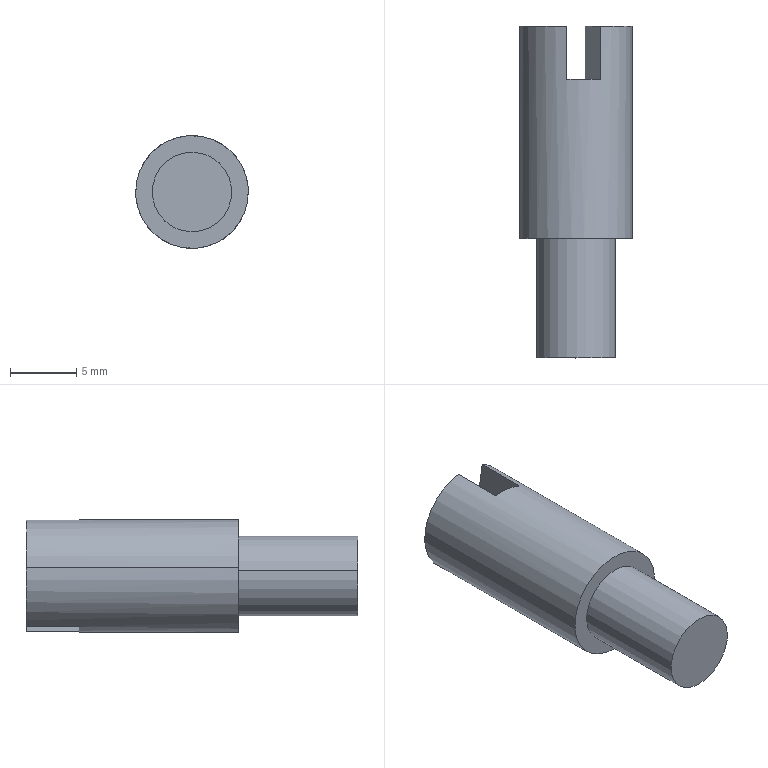Component | SolidWorks | ScrewM10X20-1 | 1 solid | 11 faces | box 8.5 x 25 x 8.5 mm | volume 1075 mm3 | plane 7 | cylinder 4 | commonest cylinder face diameters 5.993 x2 8.5 x2
build123d program:
from build123d import *

# Parameters (mm, degrees)
SKETCH1_R           = 4.25
BOSS_EXTRUDE1_DEPTH = 16
SKETCH2_R           = 2.996
BOSS_EXTRUDE2_DEPTH = 9
SKETCH3_W           = 2.587
SKETCH3_H           = 12.39
CUT_EXTRUDE1_DEPTH  = 4


with BuildPart() as part:
    # Sketch1 → Boss-Extrude1 (new body)
    with BuildSketch(Plane.XY):
        with Locations((-30.009, 15)):
            Circle(SKETCH1_R)
    extrude(amount=-BOSS_EXTRUDE1_DEPTH)

    # Sketch2 → Boss-Extrude2 (add)
    with BuildSketch(Plane(origin=(0, 0, -16), x_dir=(-1, 0, 0), z_dir=(0, 0, -1))):
        with Locations((30.009, 15)):
            Circle(SKETCH2_R)
    extrude(amount=BOSS_EXTRUDE2_DEPTH)

    # Sketch3 → Cut-Extrude1 (cut)
    with BuildSketch(Plane.XY):
        with Locations((-30.009, 15)):
            Rectangle(SKETCH3_W, SKETCH3_H)
    extrude(amount=-CUT_EXTRUDE1_DEPTH, mode=Mode.SUBTRACT)


solid = part.part

# Placed as in the assembly
solid = solid.moved(Location((1.862, 200, -4.523), (-90, 0, 8.361)))
STEP:
#1=COLOUR_RGB('',0.7922,0.8196,0.9333);
#2=FILL_AREA_STYLE_COLOUR('',#1);
#3=FILL_AREA_STYLE('',(#2));
#4=SURFACE_STYLE_FILL_AREA(#3);
#5=SURFACE_SIDE_STYLE('',(#4));
#6=SURFACE_STYLE_USAGE(.BOTH.,#5);
#7=PRESENTATION_STYLE_ASSIGNMENT((#6));
#8=CARTESIAN_POINT('',(-1.298,6.89,-0.5734));
#9=VERTEX_POINT('',#8);
#10=CARTESIAN_POINT('',(-1.065,6.89,-0.6077));
#11=VERTEX_POINT('',#10);
#12=CARTESIAN_POINT('',(-1.181,6.89,-0.5906));
#13=DIRECTION('',(0.,-1.,0.));
#14=DIRECTION('',(-0.9894,0.,0.1454));
#15=AXIS2_PLACEMENT_3D('',#12,#13,#14);
#16=CIRCLE('',#15,0.118);
#17=EDGE_CURVE('',#9,#11,#16,.T.);
#18=ORIENTED_EDGE('',*,*,#17,.F.);
#19=CARTESIAN_POINT('',(-1.298,7.244,-0.5734));
#20=VERTEX_POINT('',#19);
#21=CARTESIAN_POINT('',(-1.298,6.89,-0.5734));
#22=DIRECTION('',(0.,1.,0.));
#23=VECTOR('',#22,39.37);
#24=LINE('',#21,#23);
#25=EDGE_CURVE('',#9,#20,#24,.T.);
#26=ORIENTED_EDGE('',*,*,#25,.T.);
#27=CARTESIAN_POINT('',(-1.065,7.244,-0.6077));
#28=VERTEX_POINT('',#27);
#29=CARTESIAN_POINT('',(-1.181,7.244,-0.5906));
#30=DIRECTION('',(0.,-1.,0.));
#31=DIRECTION('',(-0.9894,0.,0.1454));
#32=AXIS2_PLACEMENT_3D('',#29,#30,#31);
#33=CIRCLE('',#32,0.118);
#34=EDGE_CURVE('',#20,#28,#33,.T.);
#35=ORIENTED_EDGE('',*,*,#34,.T.);
#36=CARTESIAN_POINT('',(-1.065,6.89,-0.6077));
#37=DIRECTION('',(0.,1.,0.));
#38=VECTOR('',#37,39.37);
#39=LINE('',#36,#38);
#40=EDGE_CURVE('',#11,#28,#39,.T.);
#41=ORIENTED_EDGE('',*,*,#40,.F.);
#42=EDGE_LOOP('',(#18,#26,#35,#41));
#43=FACE_OUTER_BOUND('',#42,.T.);
#44=CARTESIAN_POINT('',(-1.181,6.89,-0.5906));
#45=DIRECTION('',(0.,1.,0.));
#46=DIRECTION('',(0.9894,0.,-0.1454));
#47=AXIS2_PLACEMENT_3D('',#44,#45,#46);
#48=CYLINDRICAL_SURFACE('',#47,0.118);
#49=ADVANCED_FACE('',(#43),#48,.T.);
#50=CARTESIAN_POINT('',(-1.016,7.244,-0.6149));
#51=VERTEX_POINT('',#50);
#52=CARTESIAN_POINT('',(-1.347,7.244,-0.5662));
#53=VERTEX_POINT('',#52);
#54=CARTESIAN_POINT('',(-1.181,7.244,-0.5906));
#55=DIRECTION('',(0.,1.,0.));
#56=DIRECTION('',(0.9894,0.,-0.1454));
#57=AXIS2_PLACEMENT_3D('',#54,#55,#56);
#58=CIRCLE('',#57,0.1673);
#59=EDGE_CURVE('',#51,#53,#58,.T.);
#60=ORIENTED_EDGE('',*,*,#59,.T.);
#61=CARTESIAN_POINT('',(-1.347,7.874,-0.5662));
#62=VERTEX_POINT('',#61);
#63=CARTESIAN_POINT('',(-1.347,7.244,-0.5662));
#64=DIRECTION('',(0.,1.,0.));
#65=VECTOR('',#64,39.37);
#66=LINE('',#63,#65);
#67=EDGE_CURVE('',#53,#62,#66,.T.);
#68=ORIENTED_EDGE('',*,*,#67,.T.);
#69=CARTESIAN_POINT('',(-1.255,7.874,-0.7408));
#70=VERTEX_POINT('',#69);
#71=CARTESIAN_POINT('',(-1.181,7.874,-0.5906));
#72=DIRECTION('',(0.,1.,0.));
#73=DIRECTION('',(0.9894,0.,-0.1454));
#74=AXIS2_PLACEMENT_3D('',#71,#72,#73);
#75=CIRCLE('',#74,0.1673);
#76=EDGE_CURVE('',#70,#62,#75,.T.);
#77=ORIENTED_EDGE('',*,*,#76,.F.);
#78=CARTESIAN_POINT('',(-1.255,7.717,-0.7408));
#79=VERTEX_POINT('',#78);
#80=CARTESIAN_POINT('',(-1.255,7.244,-0.7408));
#81=DIRECTION('',(0.,1.,0.));
#82=VECTOR('',#81,39.37);
#83=LINE('',#80,#82);
#84=EDGE_CURVE('',#79,#70,#83,.T.);
#85=ORIENTED_EDGE('',*,*,#84,.F.);
#86=CARTESIAN_POINT('',(-1.154,7.717,-0.7556));
#87=VERTEX_POINT('',#86);
#88=CARTESIAN_POINT('',(-1.181,7.717,-0.5906));
#89=DIRECTION('',(0.,1.,0.));
#90=DIRECTION('',(-0.9894,0.,0.1454));
#91=AXIS2_PLACEMENT_3D('',#88,#89,#90);
#92=CIRCLE('',#91,0.1673);
#93=EDGE_CURVE('',#87,#79,#92,.T.);
#94=ORIENTED_EDGE('',*,*,#93,.F.);
#95=CARTESIAN_POINT('',(-1.154,7.874,-0.7556));
#96=VERTEX_POINT('',#95);
#97=CARTESIAN_POINT('',(-1.154,7.244,-0.7556));
#98=DIRECTION('',(0.,-1.,0.));
#99=VECTOR('',#98,39.37);
#100=LINE('',#97,#99);
#101=EDGE_CURVE('',#96,#87,#100,.T.);
#102=ORIENTED_EDGE('',*,*,#101,.F.);
#103=CARTESIAN_POINT('',(-1.016,7.874,-0.6149));
#104=VERTEX_POINT('',#103);
#105=CARTESIAN_POINT('',(-1.181,7.874,-0.5906));
#106=DIRECTION('',(0.,1.,0.));
#107=DIRECTION('',(0.9894,0.,-0.1454));
#108=AXIS2_PLACEMENT_3D('',#105,#106,#107);
#109=CIRCLE('',#108,0.1673);
#110=EDGE_CURVE('',#104,#96,#109,.T.);
#111=ORIENTED_EDGE('',*,*,#110,.F.);
#112=CARTESIAN_POINT('',(-1.016,7.244,-0.6149));
#113=DIRECTION('',(0.,1.,0.));
#114=VECTOR('',#113,39.37);
#115=LINE('',#112,#114);
#116=EDGE_CURVE('',#51,#104,#115,.T.);
#117=ORIENTED_EDGE('',*,*,#116,.F.);
#118=EDGE_LOOP('',(#60,#68,#77,#85,#94,#102,#111,#117));
#119=FACE_OUTER_BOUND('',#118,.T.);
#120=CARTESIAN_POINT('',(-1.181,7.244,-0.5906));
#121=DIRECTION('',(0.,1.,0.));
#122=DIRECTION('',(0.9894,0.,-0.1454));
#123=AXIS2_PLACEMENT_3D('',#120,#121,#122);
#124=CYLINDRICAL_SURFACE('',#123,0.1673);
#125=ADVANCED_FACE('',(#119),#124,.T.);
#126=CARTESIAN_POINT('',(-1.108,7.874,-0.4403));
#127=VERTEX_POINT('',#126);
#128=CARTESIAN_POINT('',(-1.131,7.874,-0.598));
#129=DIRECTION('',(-0.1454,0.,-0.9894));
#130=VECTOR('',#129,39.37);
#131=LINE('',#128,#130);
#132=EDGE_CURVE('',#127,#96,#131,.T.);
#133=ORIENTED_EDGE('',*,*,#132,.F.);
#134=CARTESIAN_POINT('',(-1.181,7.874,-0.5906));
#135=DIRECTION('',(0.,1.,0.));
#136=DIRECTION('',(0.9894,0.,-0.1454));
#137=AXIS2_PLACEMENT_3D('',#134,#135,#136);
#138=CIRCLE('',#137,0.1673);
#139=EDGE_CURVE('',#127,#104,#138,.T.);
#140=ORIENTED_EDGE('',*,*,#139,.T.);
#141=ORIENTED_EDGE('',*,*,#110,.T.);
#142=EDGE_LOOP('',(#133,#140,#141));
#143=FACE_OUTER_BOUND('',#142,.T.);
#144=CARTESIAN_POINT('',(-1.181,7.874,-0.5906));
#145=DIRECTION('',(0.,1.,0.));
#146=DIRECTION('',(0.9894,0.,-0.1454));
#147=AXIS2_PLACEMENT_3D('',#144,#145,#146);
#148=PLANE('',#147);
#149=ADVANCED_FACE('',(#143),#148,.T.);
#150=ORIENTED_EDGE('',*,*,#67,.F.);
#151=CARTESIAN_POINT('',(-1.181,7.244,-0.5906));
#152=DIRECTION('',(0.,1.,0.));
#153=DIRECTION('',(0.9894,0.,-0.1454));
#154=AXIS2_PLACEMENT_3D('',#151,#152,#153);
#155=CIRCLE('',#154,0.1673);
#156=EDGE_CURVE('',#53,#51,#155,.T.);
#157=ORIENTED_EDGE('',*,*,#156,.T.);
#158=ORIENTED_EDGE('',*,*,#116,.T.);
#159=ORIENTED_EDGE('',*,*,#139,.F.);
#160=CARTESIAN_POINT('',(-1.108,7.717,-0.4403));
#161=VERTEX_POINT('',#160);
#162=CARTESIAN_POINT('',(-1.108,7.244,-0.4403));
#163=DIRECTION('',(0.,1.,0.));
#164=VECTOR('',#163,39.37);
#165=LINE('',#162,#164);
#166=EDGE_CURVE('',#161,#127,#165,.T.);
#167=ORIENTED_EDGE('',*,*,#166,.F.);
#168=CARTESIAN_POINT('',(-1.209,7.717,-0.4255));
#169=VERTEX_POINT('',#168);
#170=CARTESIAN_POINT('',(-1.181,7.717,-0.5906));
#171=DIRECTION('',(0.,1.,0.));
#172=DIRECTION('',(-0.9894,0.,0.1454));
#173=AXIS2_PLACEMENT_3D('',#170,#171,#172);
#174=CIRCLE('',#173,0.1673);
#175=EDGE_CURVE('',#169,#161,#174,.T.);
#176=ORIENTED_EDGE('',*,*,#175,.F.);
#177=CARTESIAN_POINT('',(-1.209,7.874,-0.4255));
#178=VERTEX_POINT('',#177);
#179=CARTESIAN_POINT('',(-1.209,7.244,-0.4255));
#180=DIRECTION('',(0.,-1.,0.));
#181=VECTOR('',#180,39.37);
#182=LINE('',#179,#181);
#183=EDGE_CURVE('',#178,#169,#182,.T.);
#184=ORIENTED_EDGE('',*,*,#183,.F.);
#185=CARTESIAN_POINT('',(-1.181,7.874,-0.5906));
#186=DIRECTION('',(0.,1.,0.));
#187=DIRECTION('',(0.9894,0.,-0.1454));
#188=AXIS2_PLACEMENT_3D('',#185,#186,#187);
#189=CIRCLE('',#188,0.1673);
#190=EDGE_CURVE('',#62,#178,#189,.T.);
#191=ORIENTED_EDGE('',*,*,#190,.F.);
#192=EDGE_LOOP('',(#150,#157,#158,#159,#167,#176,#184,#191));
#193=FACE_OUTER_BOUND('',#192,.T.);
#194=CARTESIAN_POINT('',(-1.181,7.244,-0.5906));
#195=DIRECTION('',(0.,1.,0.));
#196=DIRECTION('',(0.9894,0.,-0.1454));
#197=AXIS2_PLACEMENT_3D('',#194,#195,#196);
#198=CYLINDRICAL_SURFACE('',#197,0.1673);
#199=ADVANCED_FACE('',(#193),#198,.T.);
#200=CARTESIAN_POINT('',(-1.181,7.244,-0.5906));
#201=DIRECTION('',(0.,-1.,0.));
#202=DIRECTION('',(-0.9894,0.,0.1454));
#203=AXIS2_PLACEMENT_3D('',#200,#201,#202);
#204=CIRCLE('',#203,0.118);
#205=EDGE_CURVE('',#28,#20,#204,.T.);
#206=ORIENTED_EDGE('',*,*,#205,.F.);
#207=ORIENTED_EDGE('',*,*,#34,.F.);
#208=EDGE_LOOP('',(#206,#207));
#209=FACE_BOUND('',#208,.T.);
#210=ORIENTED_EDGE('',*,*,#59,.F.);
#211=ORIENTED_EDGE('',*,*,#156,.F.);
#212=EDGE_LOOP('',(#210,#211));
#213=FACE_OUTER_BOUND('',#212,.T.);
#214=CARTESIAN_POINT('',(-1.181,7.244,-0.5906));
#215=DIRECTION('',(0.,1.,0.));
#216=DIRECTION('',(0.9894,0.,-0.1454));
#217=AXIS2_PLACEMENT_3D('',#214,#215,#216);
#218=PLANE('',#217);
#219=ADVANCED_FACE('',(#209,#213),#218,.F.);
#220=CARTESIAN_POINT('',(-1.232,7.874,-0.5831));
#221=DIRECTION('',(0.1454,0.,0.9894));
#222=VECTOR('',#221,39.37);
#223=LINE('',#220,#222);
#224=EDGE_CURVE('',#70,#178,#223,.T.);
#225=ORIENTED_EDGE('',*,*,#224,.F.);
#226=ORIENTED_EDGE('',*,*,#76,.T.);
#227=ORIENTED_EDGE('',*,*,#190,.T.);
#228=EDGE_LOOP('',(#225,#226,#227));
#229=FACE_OUTER_BOUND('',#228,.T.);
#230=CARTESIAN_POINT('',(-1.181,7.874,-0.5906));
#231=DIRECTION('',(0.,1.,0.));
#232=DIRECTION('',(0.9894,0.,-0.1454));
#233=AXIS2_PLACEMENT_3D('',#230,#231,#232);
#234=PLANE('',#233);
#235=ADVANCED_FACE('',(#229),#234,.T.);
#236=ORIENTED_EDGE('',*,*,#25,.F.);
#237=CARTESIAN_POINT('',(-1.181,6.89,-0.5906));
#238=DIRECTION('',(0.,-1.,0.));
#239=DIRECTION('',(-0.9894,0.,0.1454));
#240=AXIS2_PLACEMENT_3D('',#237,#238,#239);
#241=CIRCLE('',#240,0.118);
#242=EDGE_CURVE('',#11,#9,#241,.T.);
#243=ORIENTED_EDGE('',*,*,#242,.F.);
#244=ORIENTED_EDGE('',*,*,#40,.T.);
#245=ORIENTED_EDGE('',*,*,#205,.T.);
#246=EDGE_LOOP('',(#236,#243,#244,#245));
#247=FACE_OUTER_BOUND('',#246,.T.);
#248=CARTESIAN_POINT('',(-1.181,6.89,-0.5906));
#249=DIRECTION('',(0.,1.,0.));
#250=DIRECTION('',(0.9894,0.,-0.1454));
#251=AXIS2_PLACEMENT_3D('',#248,#249,#250);
#252=CYLINDRICAL_SURFACE('',#251,0.118);
#253=ADVANCED_FACE('',(#247),#252,.T.);
#254=ORIENTED_EDGE('',*,*,#242,.T.);
#255=ORIENTED_EDGE('',*,*,#17,.T.);
#256=EDGE_LOOP('',(#254,#255));
#257=FACE_OUTER_BOUND('',#256,.T.);
#258=CARTESIAN_POINT('',(-1.181,6.89,-0.5906));
#259=DIRECTION('',(0.,-1.,0.));
#260=DIRECTION('',(-0.9894,0.,0.1454));
#261=AXIS2_PLACEMENT_3D('',#258,#259,#260);
#262=PLANE('',#261);
#263=ADVANCED_FACE('',(#257),#262,.T.);
#264=ORIENTED_EDGE('',*,*,#101,.T.);
#265=CARTESIAN_POINT('',(-1.096,7.717,-0.3566));
#266=DIRECTION('',(-0.1454,0.,-0.9894));
#267=VECTOR('',#266,39.37);
#268=LINE('',#265,#267);
#269=EDGE_CURVE('',#161,#87,#268,.T.);
#270=ORIENTED_EDGE('',*,*,#269,.F.);
#271=ORIENTED_EDGE('',*,*,#166,.T.);
#272=ORIENTED_EDGE('',*,*,#132,.T.);
#273=EDGE_LOOP('',(#264,#270,#271,#272));
#274=FACE_OUTER_BOUND('',#273,.T.);
#275=CARTESIAN_POINT('',(-1.096,7.717,-0.3566));
#276=DIRECTION('',(0.9894,0.,-0.1454));
#277=DIRECTION('',(0.,-1.,0.));
#278=AXIS2_PLACEMENT_3D('',#275,#276,#277);
#279=PLANE('',#278);
#280=ADVANCED_FACE('',(#274),#279,.F.);
#281=ORIENTED_EDGE('',*,*,#183,.T.);
#282=CARTESIAN_POINT('',(-1.196,7.717,-0.3418));
#283=DIRECTION('',(0.1454,0.,0.9894));
#284=VECTOR('',#283,39.37);
#285=LINE('',#282,#284);
#286=EDGE_CURVE('',#79,#169,#285,.T.);
#287=ORIENTED_EDGE('',*,*,#286,.F.);
#288=ORIENTED_EDGE('',*,*,#84,.T.);
#289=ORIENTED_EDGE('',*,*,#224,.T.);
#290=EDGE_LOOP('',(#281,#287,#288,#289));
#291=FACE_OUTER_BOUND('',#290,.T.);
#292=CARTESIAN_POINT('',(-1.196,7.717,-0.3418));
#293=DIRECTION('',(-0.9894,0.,0.1454));
#294=DIRECTION('',(0.,1.,0.));
#295=AXIS2_PLACEMENT_3D('',#292,#293,#294);
#296=PLANE('',#295);
#297=ADVANCED_FACE('',(#291),#296,.F.);
#298=ORIENTED_EDGE('',*,*,#175,.T.);
#299=ORIENTED_EDGE('',*,*,#269,.T.);
#300=ORIENTED_EDGE('',*,*,#93,.T.);
#301=ORIENTED_EDGE('',*,*,#286,.T.);
#302=EDGE_LOOP('',(#298,#299,#300,#301));
#303=FACE_OUTER_BOUND('',#302,.T.);
#304=CARTESIAN_POINT('',(0.07331,7.717,-0.1781));
#305=DIRECTION('',(0.,-1.,0.));
#306=DIRECTION('',(-0.9894,0.,0.1454));
#307=AXIS2_PLACEMENT_3D('',#304,#305,#306);
#308=PLANE('',#307);
#309=ADVANCED_FACE('',(#303),#308,.F.);
#310=CLOSED_SHELL('',(#49,#125,#149,#199,#219,#235,#253,#263,#280,#297,#309));
#311=MANIFOLD_SOLID_BREP('',#310);
#312=STYLED_ITEM('',(#7),#311);
#313=PRESENTATION_LAYER_ASSIGNMENT('','',(#312));
#314=CARTESIAN_POINT('',(0.,0.,0.));
#315=DIRECTION('',(0.,0.,1.));
#316=DIRECTION('',(1.,0.,0.));
#317=AXIS2_PLACEMENT_3D('',#314,#315,#316);
#318=(LENGTH_UNIT()NAMED_UNIT(*)SI_UNIT($,.METRE.));
#319=LENGTH_MEASURE_WITH_UNIT(LENGTH_MEASURE(0.0254),#318);
#320=DIMENSIONAL_EXPONENTS(1.,0.,0.,0.,0.,0.,0.);
#321=(CONVERSION_BASED_UNIT('',#319)LENGTH_UNIT()NAMED_UNIT(#320));
#322=UNCERTAINTY_MEASURE_WITH_UNIT(LENGTH_MEASURE(0.00001),#321,'','');
#323=(NAMED_UNIT(*)PLANE_ANGLE_UNIT()SI_UNIT($,.RADIAN.));
#324=(NAMED_UNIT(*)SI_UNIT($,.STERADIAN.)SOLID_ANGLE_UNIT());
#325=(GEOMETRIC_REPRESENTATION_CONTEXT(3)GLOBAL_UNCERTAINTY_ASSIGNED_CONTEXT((#322))GLOBAL_UNIT_ASSIGNED_CONTEXT((#321,#323,#324))REPRESENTATION_CONTEXT('',''));
#326=ADVANCED_BREP_SHAPE_REPRESENTATION('',(#311,#317),#325);
#327=(LENGTH_UNIT()NAMED_UNIT(*)SI_UNIT($,.METRE.));
#328=LENGTH_MEASURE_WITH_UNIT(LENGTH_MEASURE(0.0254),#327);
#329=DIMENSIONAL_EXPONENTS(1.,0.,0.,0.,0.,0.,0.);
#330=(CONVERSION_BASED_UNIT('',#328)LENGTH_UNIT()NAMED_UNIT(#329));
#331=UNCERTAINTY_MEASURE_WITH_UNIT(LENGTH_MEASURE(0.00001),#330,'','');
#332=(NAMED_UNIT(*)PLANE_ANGLE_UNIT()SI_UNIT($,.RADIAN.));
#333=(NAMED_UNIT(*)SI_UNIT($,.STERADIAN.)SOLID_ANGLE_UNIT());
#334=(GEOMETRIC_REPRESENTATION_CONTEXT(3)GLOBAL_UNCERTAINTY_ASSIGNED_CONTEXT((#331))GLOBAL_UNIT_ASSIGNED_CONTEXT((#330,#332,#333))REPRESENTATION_CONTEXT('',''));
#335=MECHANICAL_DESIGN_GEOMETRIC_PRESENTATION_REPRESENTATION('',(#312),#334);